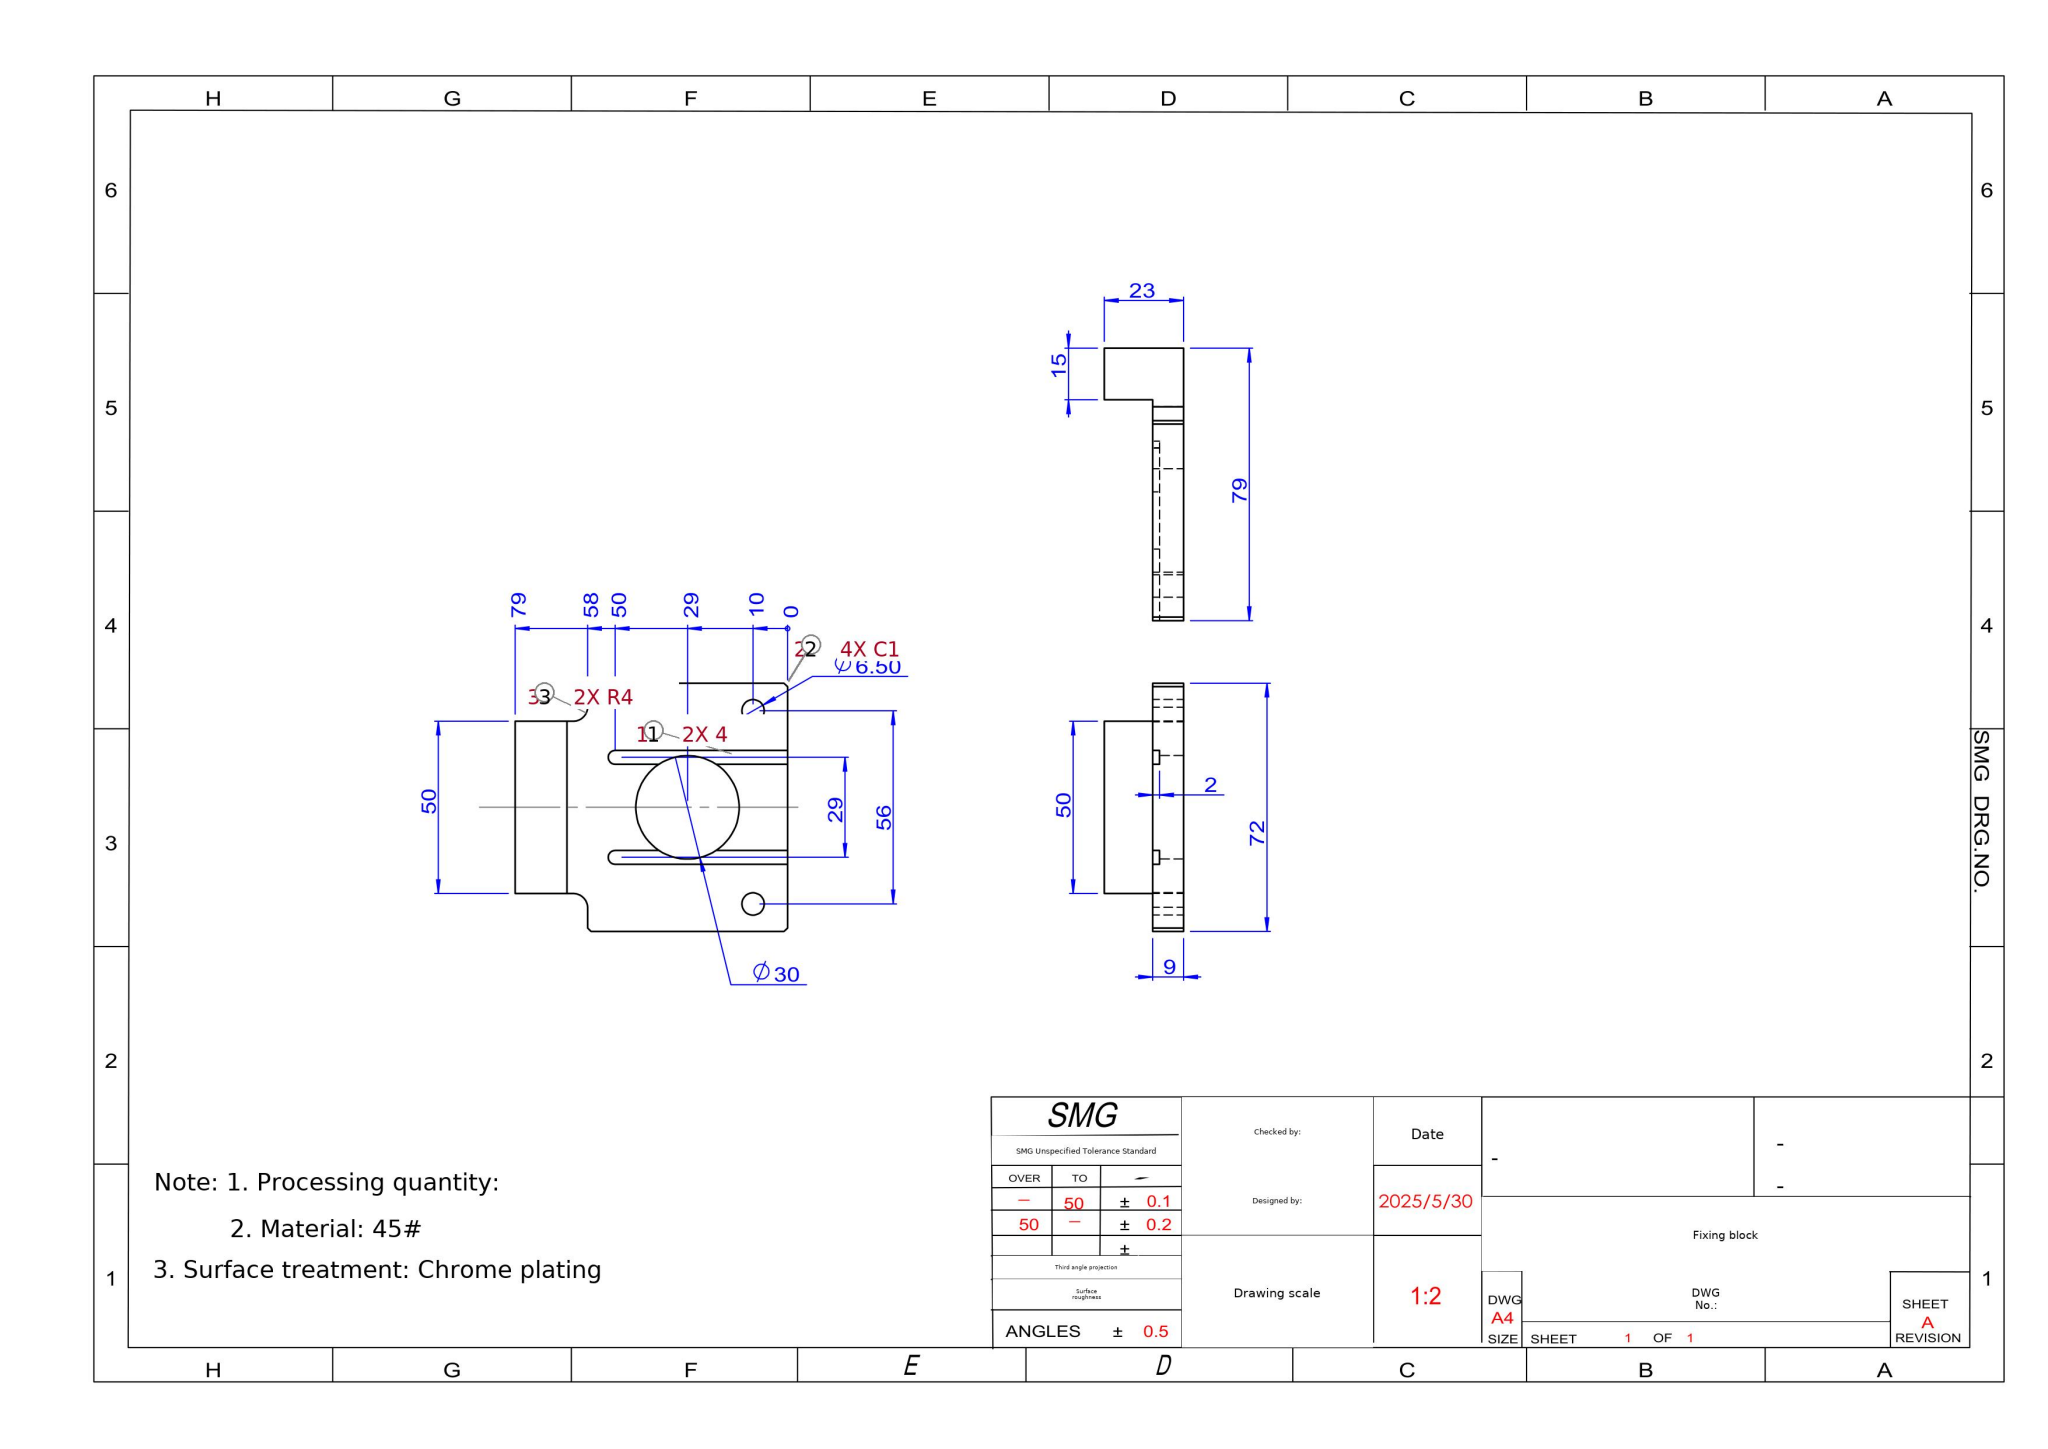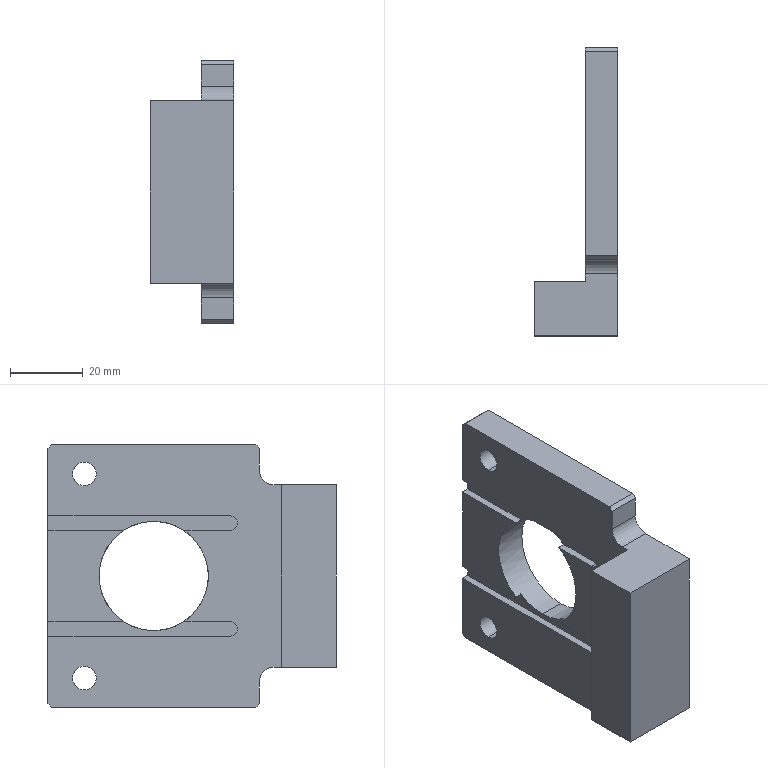Part | SolidWorks | mm | material 45# | 1 solid | 37 faces | box 23 x 79 x 72 mm | volume 49906 mm3 | plane 25 | cylinder 12 | commonest cylinder face diameters 6.5 x4 4 x4 30 x2 8 x2